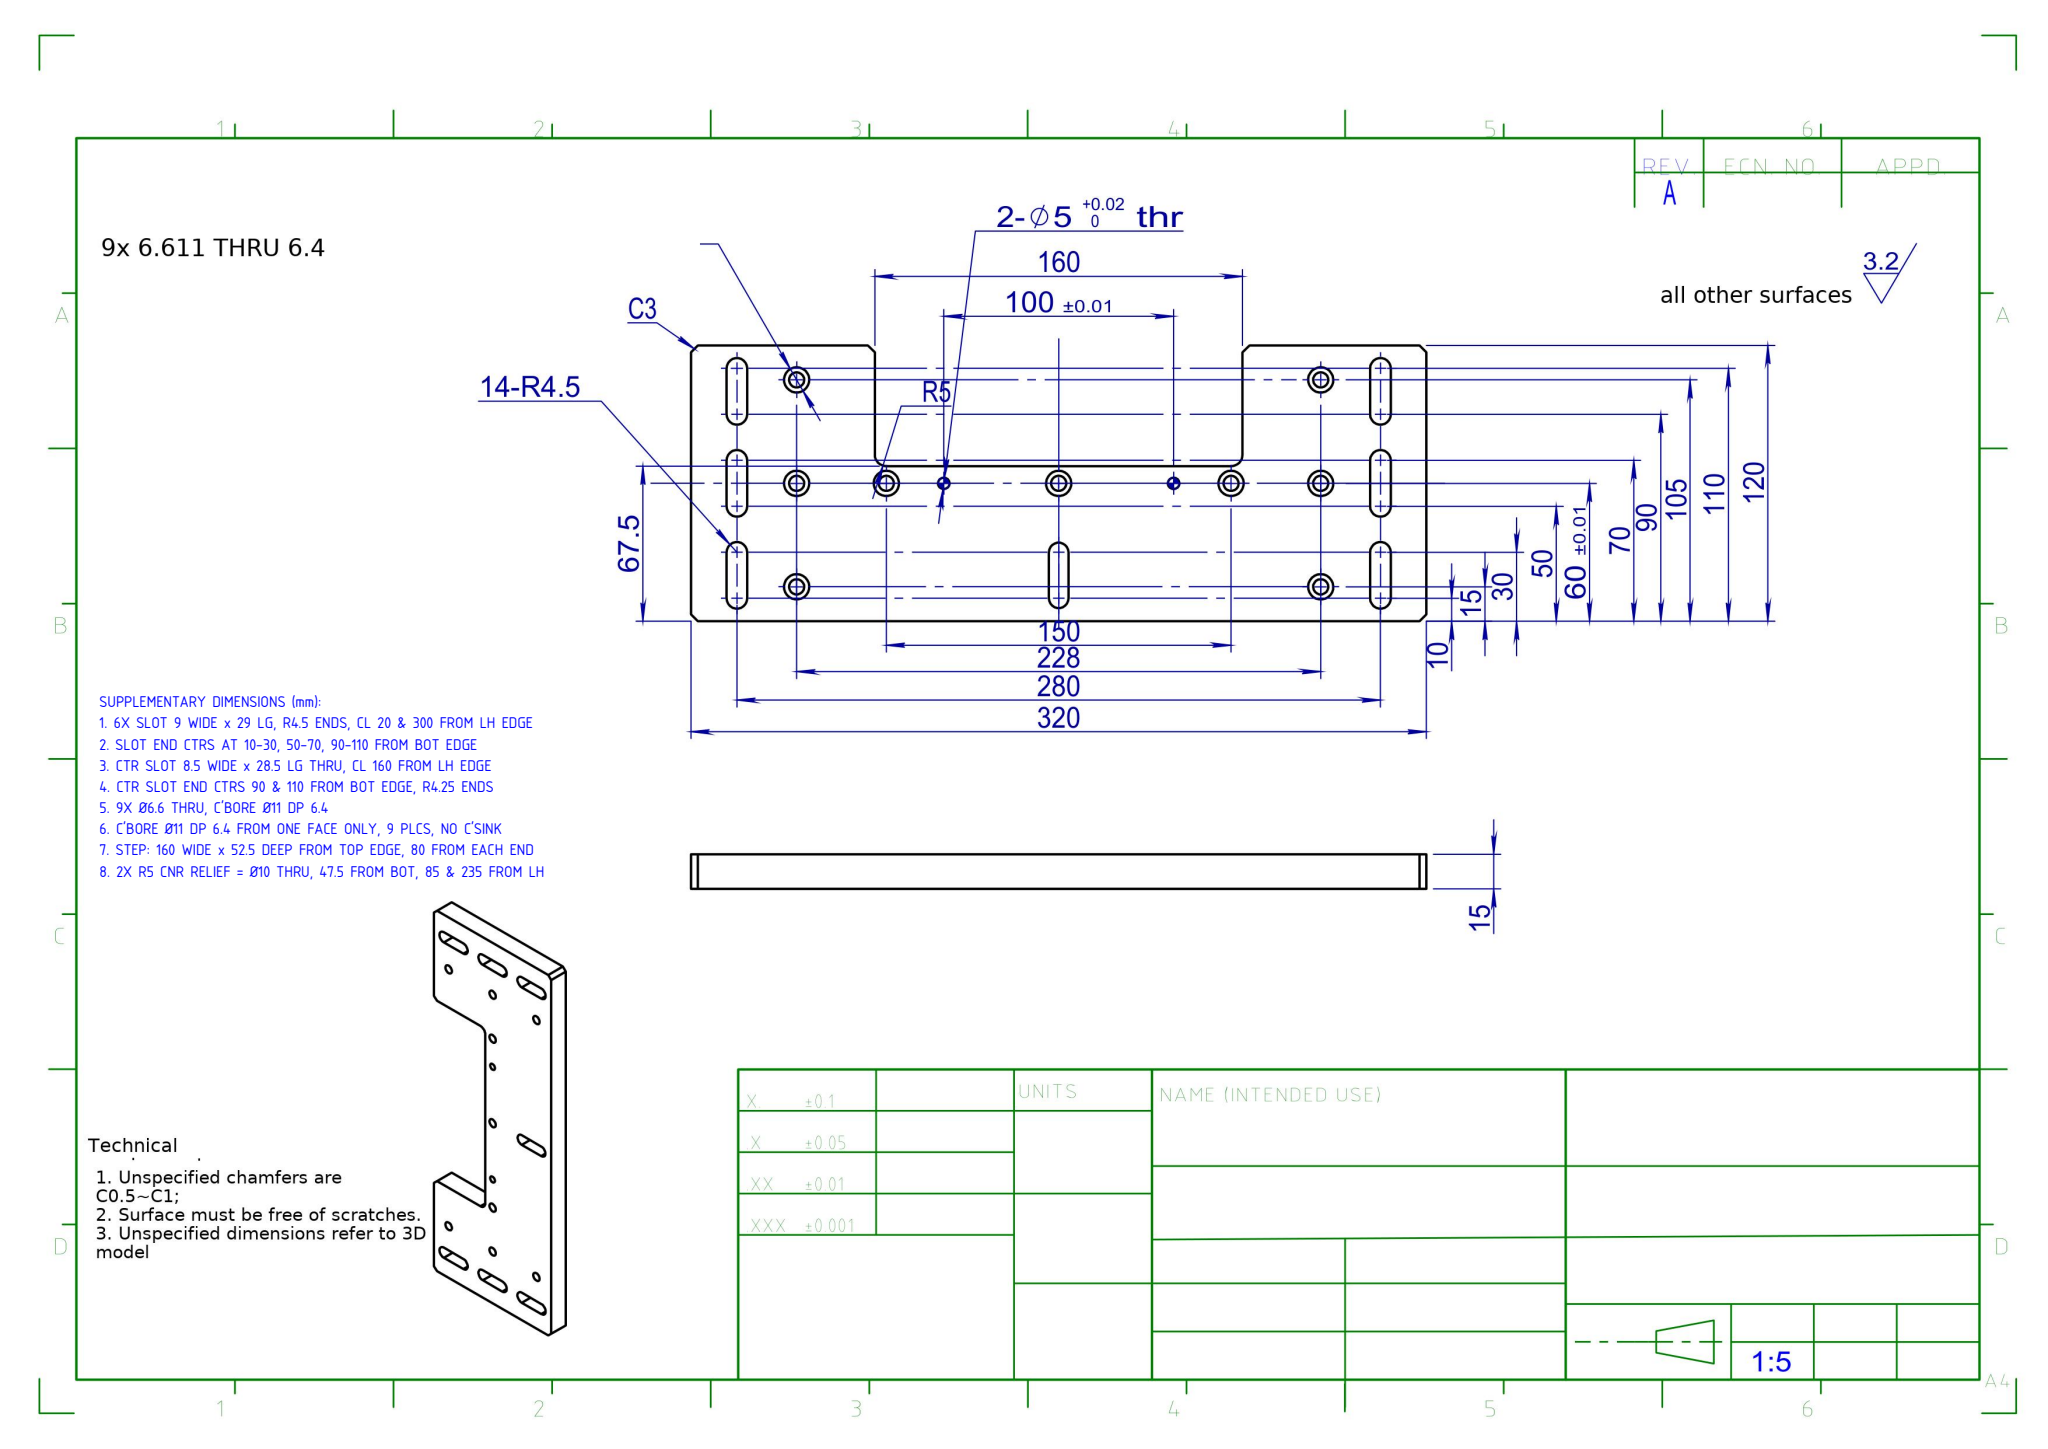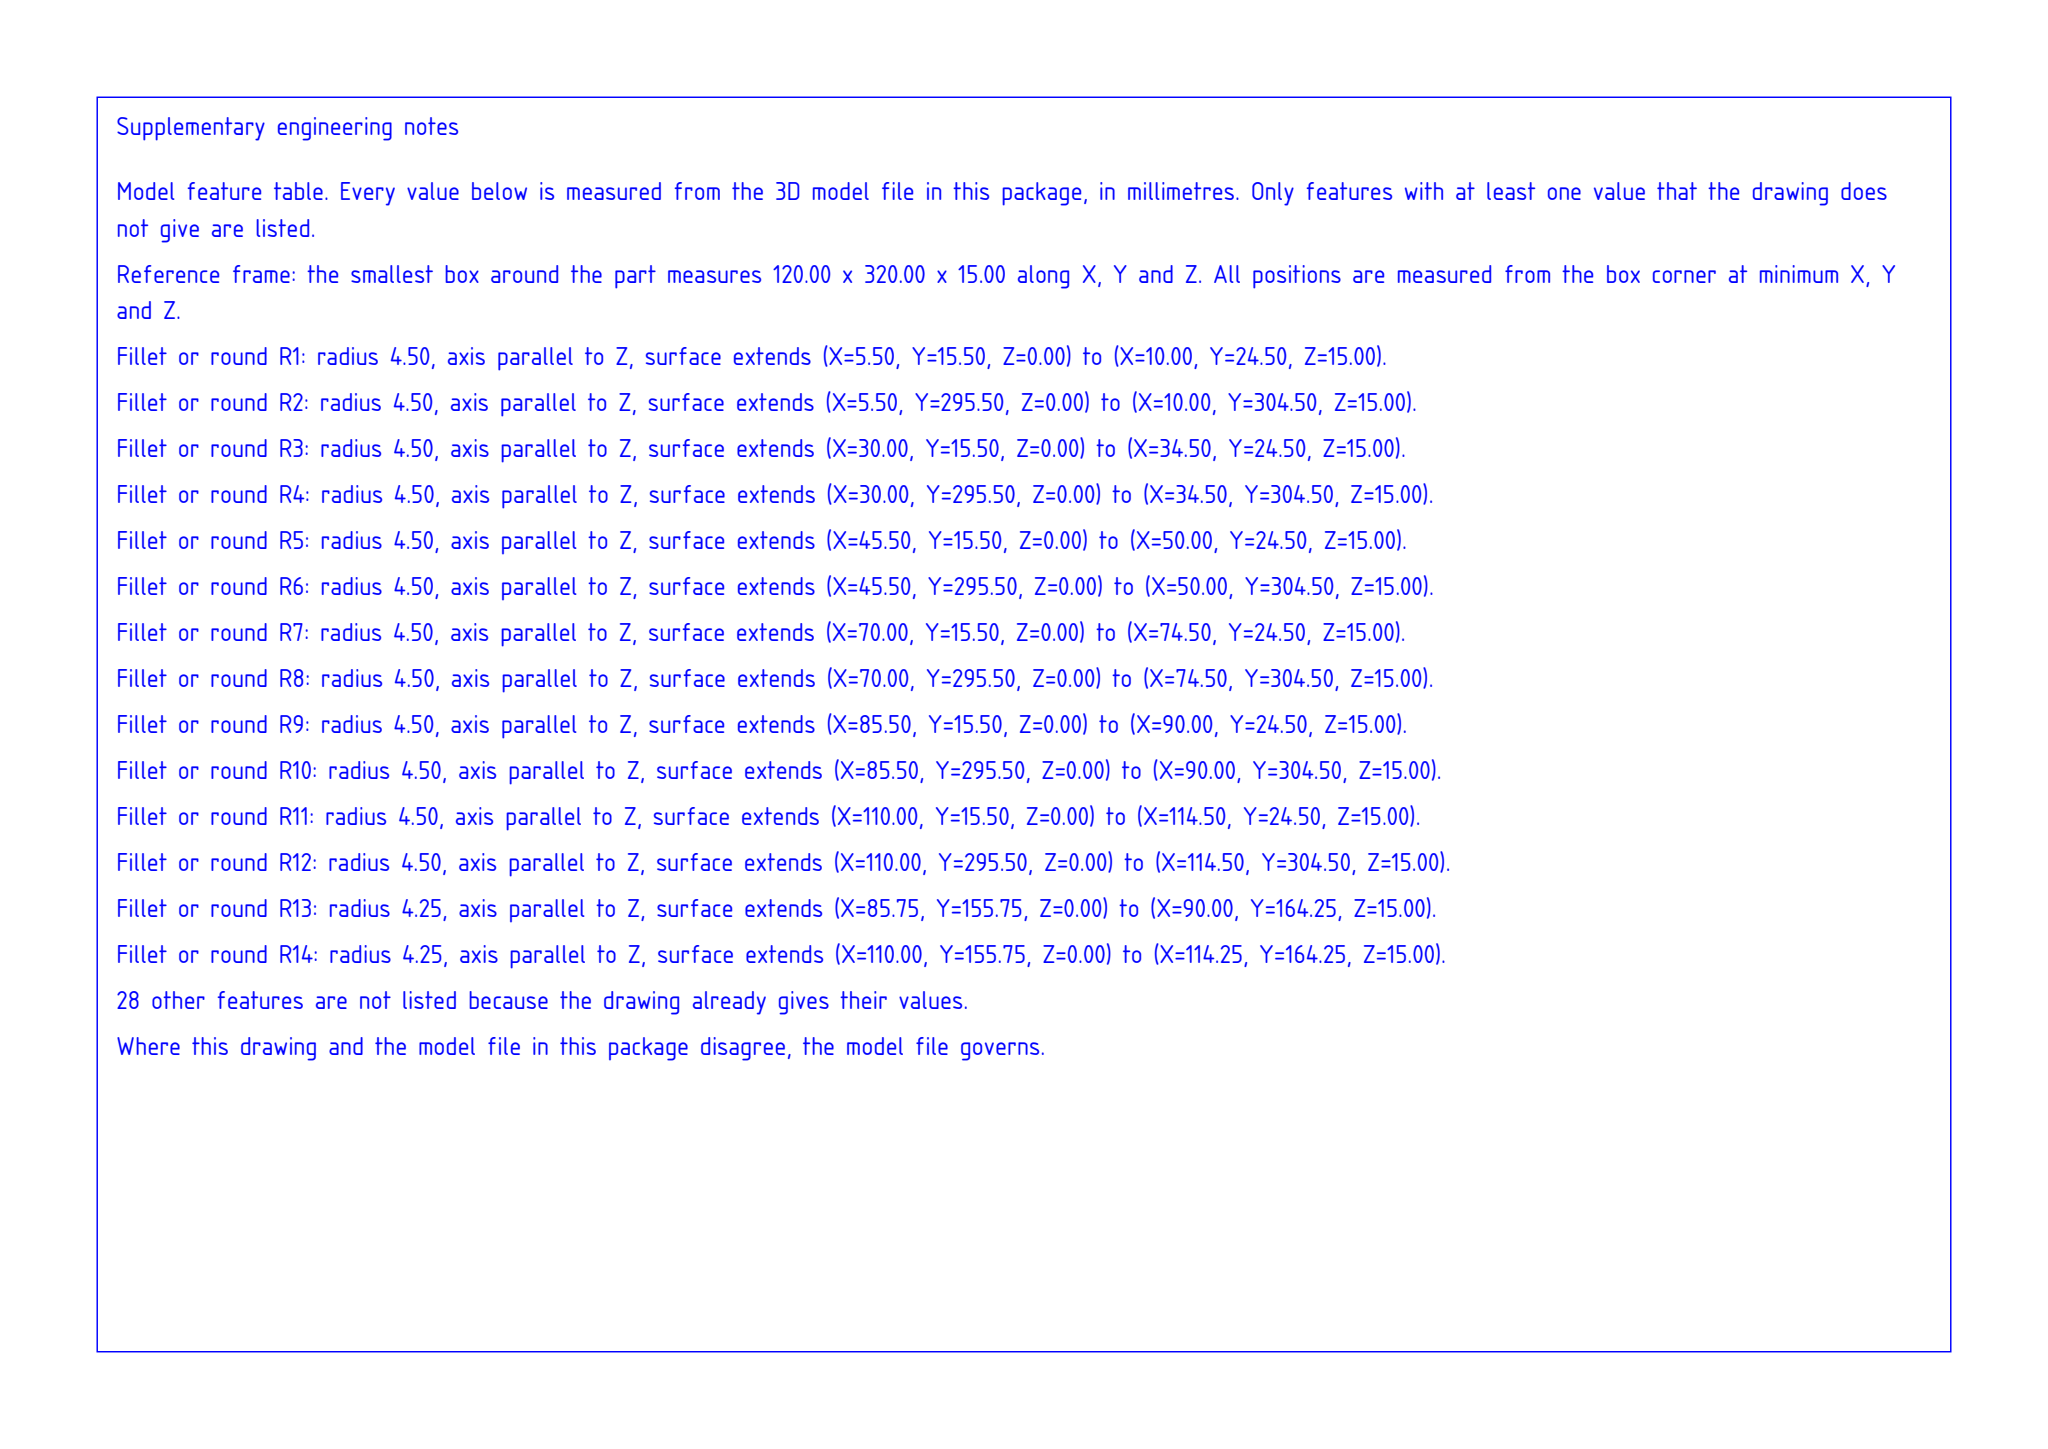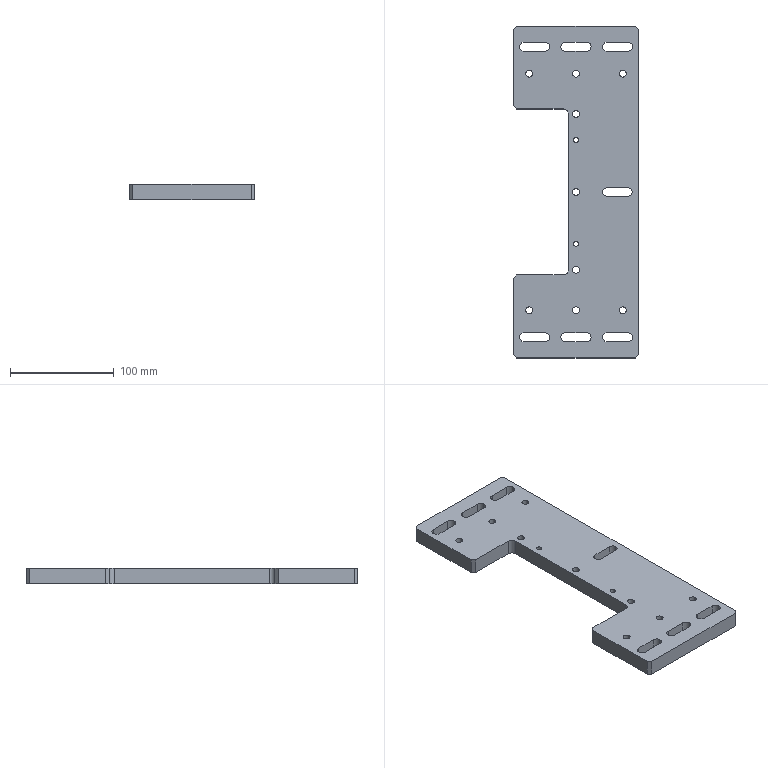Part | SolidWorks | mm | 1 solid | 102 faces | box 120 x 320 x 15 mm | volume 415718 mm3 | cylinder 63 | plane 39 | commonest cylinder face diameters 11 x18 6.6 x18 9 x18 5 x4 8.5 x3 10 x2
build123d program:
from build123d import *

# Parameters (mm, degrees)
SKETCH1_W                                            = 60
SKETCH1_H                                            = 320
BOSS_EXTRUDE1_DEPTH                                  = 15
SKETCH1_2_W                                          = 60
SKETCH1_2_H                                          = 80
BOSS_EXTRUDE1_2_DEPTH                                = 15
CUT_EXTRUDE1_DEPTH                                   = 185.187
SKETCH3_W                                            = 15
SKETCH3_H                                            = 160
BOSS_EXTRUDE2_DEPTH                                  = 7.5
FILLET1_R                                            = 5
CUT_EXTRUDE5_DEPTH                                   = 185.187
M6_HEX_SOCKET_HEAD_CAP_SCREW_COUNTERBORE_D           = 6.6
M6_HEX_SOCKET_HEAD_CAP_SCREW_COUNTERBORE_CBORE_D     = 11
M6_HEX_SOCKET_HEAD_CAP_SCREW_COUNTERBORE_CBORE_DEPTH = 6.4
M6_HEX_SOCKET_HEAD_CAP_SCREW_COUNTER_2_D             = 6.6
M6_HEX_SOCKET_HEAD_CAP_SCREW_COUNTER_2_CBORE_D       = 11
M6_HEX_SOCKET_HEAD_CAP_SCREW_COUNTER_2_CBORE_DEPTH   = 6.4
SKETCH10_R                                           = 2.5
CUT_EXTRUDE6_DEPTH                                   = 185.187
CHAMFER1_SIZE                                        = 3


with BuildPart() as part:
    # Sketch1 → Boss-Extrude1 (new body)
    with BuildSketch(Plane.XY):
        Rectangle(SKETCH1_W, SKETCH1_H)
    extrude(amount=BOSS_EXTRUDE1_DEPTH)

    # Sketch1_2 → Boss-Extrude1_2 (add)
    with BuildSketch(Plane.XY.offset(15)):
        with Locations((-60, 120)):
            Rectangle(SKETCH1_2_W, SKETCH1_2_H)
        with Locations((-60, -120)):
            Rectangle(SKETCH1_2_W, SKETCH1_2_H)
    extrude(amount=-BOSS_EXTRUDE1_2_DEPTH)

    # Sketch2 → Cut-Extrude1 (cut, through all)
    with BuildSketch(Plane.XY.offset(15)):
        with BuildLine():
            Line((-80, -135.5), (-60, -135.5))
            ThreePointArc((-60, -135.5), (-55.5, -140), (-60, -144.5))
            Line((-60, -144.5), (-80, -144.5))
            ThreePointArc((-80, -144.5), (-84.5, -140), (-80, -135.5))
        make_face()
        with BuildLine():
            Line((0, -135.5), (20, -135.5))
            ThreePointArc((20, -135.5), (24.5, -140), (20, -144.5))
            Line((20, -144.5), (0, -144.5))
            ThreePointArc((0, -144.5), (-4.5, -140), (0, -135.5))
        make_face()
        with BuildLine():
            Line((-40, -135.5), (-20, -135.5))
            ThreePointArc((-20, -135.5), (-15.5, -140), (-20, -144.5))
            Line((-20, -144.5), (-40, -144.5))
            ThreePointArc((-40, -144.5), (-44.5, -140), (-40, -135.5))
        make_face()
    cut_extrude1 = extrude(amount=-CUT_EXTRUDE1_DEPTH, mode=Mode.SUBTRACT)

    # Mirror1: Cut-Extrude1 across plane
    add(cut_extrude1.mirror(Plane.ZX), mode=Mode.SUBTRACT)

    # Sketch3 → Boss-Extrude2 (add)
    with BuildSketch(Plane.ZY.offset(30)):
        with Locations((7.5, 0)):
            Rectangle(SKETCH3_W, SKETCH3_H)
    extrude(amount=BOSS_EXTRUDE2_DEPTH)

    # Fillet1
    fillet1_edges = [part.edges().sort_by_distance(p)[0] for p in [
        (-37.5, -80, 7.5),
        (-37.5, 80, 7.5),
    ]]
    fillet(fillet1_edges, radius=FILLET1_R)

    # Sketch5 → Cut-Extrude5 (cut, through all)
    with BuildSketch(Plane.XY.offset(15)):
        with BuildLine():
            Line((0, 4.25), (20, 4.25))
            ThreePointArc((20, 4.25), (24.25, 0), (20, -4.25))
            Line((20, -4.25), (0, -4.25))
            ThreePointArc((0, -4.25), (-4.25, 0), (0, 4.25))
        make_face()
    extrude(amount=-CUT_EXTRUDE5_DEPTH, mode=Mode.SUBTRACT)

    # M6 Hex Socket Head Cap Screw Counterbore (through all)
    with Locations(Plane(origin=(0, 0, 0), x_dir=(-1, 0, 0), z_dir=(0, 0, -1))):
        with Locations((-15, -114), (30, -114), (75, -114)):
            m6_hex_socket_head_cap_screw_counterbore = CounterBoreHole(M6_HEX_SOCKET_HEAD_CAP_SCREW_COUNTERBORE_D / 2, M6_HEX_SOCKET_HEAD_CAP_SCREW_COUNTERBORE_CBORE_D / 2, M6_HEX_SOCKET_HEAD_CAP_SCREW_COUNTERBORE_CBORE_DEPTH)

    # Mirror2: M6 Hex Socket Head Cap Screw Counterbore across plane
    add(m6_hex_socket_head_cap_screw_counterbore.mirror(Plane.ZX), mode=Mode.SUBTRACT)

    # M6 Hex Socket Head Cap Screw Counter 2 (through all)
    with Locations(Plane(origin=(0, 0, 0), x_dir=(-1, 0, 0), z_dir=(0, 0, -1))):
        with Locations((30, 0), (30, -75), (30, 75)):
            CounterBoreHole(M6_HEX_SOCKET_HEAD_CAP_SCREW_COUNTER_2_D / 2, M6_HEX_SOCKET_HEAD_CAP_SCREW_COUNTER_2_CBORE_D / 2, M6_HEX_SOCKET_HEAD_CAP_SCREW_COUNTER_2_CBORE_DEPTH)

    # Sketch10 → Cut-Extrude6 (cut, through all)
    with BuildSketch(Plane(origin=(0, 0, 0), x_dir=(-1, 0, 0), z_dir=(0, 0, -1))):
        with Locations((30, -50)):
            Circle(SKETCH10_R)
        with Locations((30, 50)):
            Circle(SKETCH10_R)
    extrude(amount=-CUT_EXTRUDE6_DEPTH, mode=Mode.SUBTRACT)

    # Chamfer1
    chamfer1_edges = [part.edges().sort_by_distance(p)[0] for p in [
        (30, 160, 7.5),
        (-90, 160, 7.5),
        (-90, 80, 7.5),
        (-90, -80, 7.5),
        (-90, -160, 7.5),
        (30, -160, 7.5),
    ]]
    chamfer(chamfer1_edges, length=CHAMFER1_SIZE)


solid = part.part